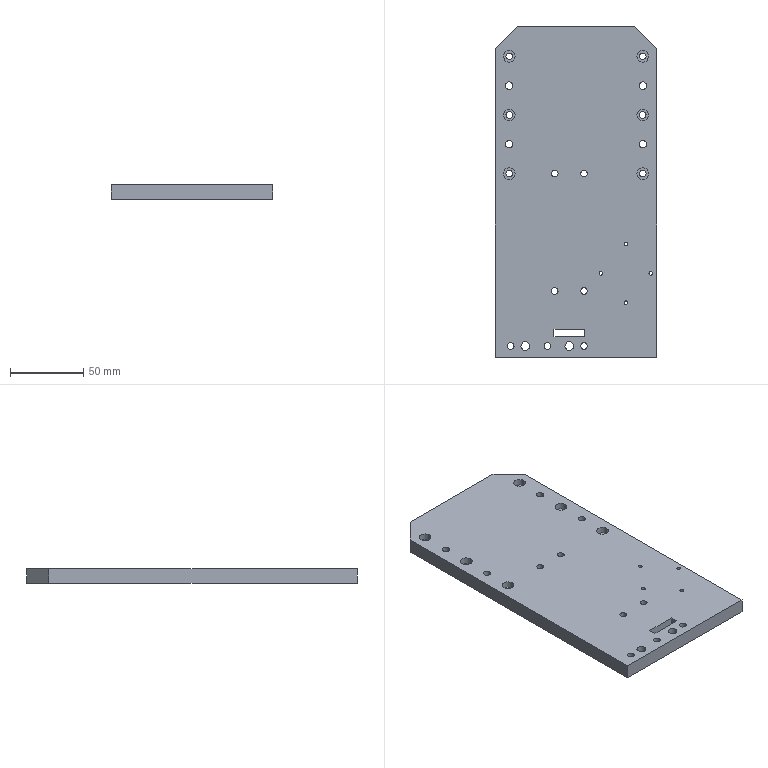Component | SolidWorks | GbgbYAxisConnectionPlate-1 | 1 solid | 97 faces | box 110 x 225 x 10 mm | volume 238530 mm3 | cylinder 72 | plane 25 | commonest cylinder face diameters 8 x26 4.5 x26 5 x8 2.5 x8 6 x4 | material AL6061
build123d program:
from build123d import *

# Parameters (mm, degrees)
SKETCH1_W                                            = 110
SKETCH1_H                                            = 220
BOSS_EXTRUDE1_DEPTH                                  = 5
M3_TAPPED_HOLE1_D                                    = 2.5
HOLE_SIZE_ACCORDING_TO_THE_TYPE_OF_HEX_S_D           = 4.5
HOLE_SIZE_ACCORDING_TO_THE_TYPE_OF_HEX_S_CBORE_D     = 8
HOLE_SIZE_ACCORDING_TO_THE_TYPE_OF_HEX_S_CBORE_DEPTH = 4.6
LPATTERN1_COUNT                                      = 3
LPATTERN1_PITCH                                      = 40
SKETCH13_W                                           = 21
SKETCH13_H                                           = 5
CUT_EXTRUDE2_DEPTH                                   = 10
MOVE_FACE1_BY                                        = 5
HOLE_SIZE_ACCORDING_TO_THE_TYPE_OF_H_2_D             = 4.5
HOLE_SIZE_ACCORDING_TO_THE_TYPE_OF_H_2_CBORE_D       = 8
HOLE_SIZE_ACCORDING_TO_THE_TYPE_OF_H_2_CBORE_DEPTH   = 4.6
HOLE_SIZE_ACCORDING_TO_THE_TYPE_OF_H_3_D             = 4.5
HOLE_SIZE_ACCORDING_TO_THE_TYPE_OF_H_3_CBORE_D       = 8
HOLE_SIZE_ACCORDING_TO_THE_TYPE_OF_H_3_CBORE_DEPTH   = 4.6
SKETCH20_R                                           = 3
CUT_EXTRUDE3_DEPTH                                   = 128.867
SKETCH21_R                                           = 2.5
CUT_EXTRUDE4_DEPTH                                   = 15
LPATTERN2_COUNT                                      = 2
LPATTERN2_PITCH                                      = 40
CHAMFER1_SIZE                                        = 15


with BuildPart() as part:
    # Sketch1 → Boss-Extrude1 (new, symmetric)
    with BuildSketch(Plane.XY):
        Rectangle(SKETCH1_W, SKETCH1_H)
    extrude(amount=BOSS_EXTRUDE1_DEPTH, both=True)

    # M3 Tapped Hole1 (through all)
    with Locations(Plane.XY.offset(5)):
        with Locations((34, -38), (17, -58), (51, -58), (34, -78)):
            Hole(M3_TAPPED_HOLE1_D / 2)

    # Hole Size according to the type of hex s (through all)
    with Locations(Plane.XY.offset(5)):
        with Locations((-45.5, 90), (45.5, 90)):
            hole_size_according_to_the_type_of_hex_s = CounterBoreHole(HOLE_SIZE_ACCORDING_TO_THE_TYPE_OF_HEX_S_D / 2, HOLE_SIZE_ACCORDING_TO_THE_TYPE_OF_HEX_S_CBORE_D / 2, HOLE_SIZE_ACCORDING_TO_THE_TYPE_OF_HEX_S_CBORE_DEPTH)

    # LPattern1: Hole Size according to the type of hex s ×3
    with Locations(*[(0, -i * LPATTERN1_PITCH, 0) for i in range(1, LPATTERN1_COUNT)]):
        add(hole_size_according_to_the_type_of_hex_s, mode=Mode.SUBTRACT)

    # Sketch13 → Cut-Extrude2 (cut)
    with BuildSketch(Plane(origin=(0, 0, -5), x_dir=(-1, 0, 0), z_dir=(0, 0, -1))):
        with Locations((4.5, -98.6)):
            Rectangle(SKETCH13_W, SKETCH13_H)
    extrude(amount=-CUT_EXTRUDE2_DEPTH, mode=Mode.SUBTRACT)

    # Move Face1: a face moved outward by 5.0
    extrude(part.faces().sort_by_distance((0, -110, 0))[0], amount=MOVE_FACE1_BY, dir=(0, -1, 0))

    # Hole Size according to the type of h 2 (through all)
    with Locations(Plane(origin=(0, 0, -5), x_dir=(-1, 0, 0), z_dir=(0, 0, -1))):
        with Locations((44.5, -107.5), (19.5, -107.5), (-5.5, -107.5)):
            CounterBoreHole(HOLE_SIZE_ACCORDING_TO_THE_TYPE_OF_H_2_D / 2, HOLE_SIZE_ACCORDING_TO_THE_TYPE_OF_H_2_CBORE_D / 2, HOLE_SIZE_ACCORDING_TO_THE_TYPE_OF_H_2_CBORE_DEPTH)

    # Hole Size according to the type of h 3 (through all)
    with Locations(Plane(origin=(0, 0, -5), x_dir=(-1, 0, 0), z_dir=(0, 0, -1))):
        with Locations((-5.5, -70), (14.5, -70), (-5.5, 10), (14.5, 10)):
            CounterBoreHole(HOLE_SIZE_ACCORDING_TO_THE_TYPE_OF_H_3_D / 2, HOLE_SIZE_ACCORDING_TO_THE_TYPE_OF_H_3_CBORE_D / 2, HOLE_SIZE_ACCORDING_TO_THE_TYPE_OF_H_3_CBORE_DEPTH)

    # Sketch20 → Cut-Extrude3 (cut, through all)
    with BuildSketch(Plane(origin=(0, 0, -5), x_dir=(-1, 0, 0), z_dir=(0, 0, -1))):
        with Locations((4.5, -107.5)):
            Circle(SKETCH20_R)
        with Locations((34.5, -107.5)):
            Circle(SKETCH20_R)
    extrude(amount=-CUT_EXTRUDE3_DEPTH, mode=Mode.SUBTRACT)

    # Sketch21 → Cut-Extrude4 (cut)
    with BuildSketch(Plane.XY.offset(5)):
        with Locations((-45.5, 70)):
            Circle(SKETCH21_R)
        with Locations((45.5, 70)):
            Circle(SKETCH21_R)
    cut_extrude4 = extrude(amount=-CUT_EXTRUDE4_DEPTH, mode=Mode.SUBTRACT)

    # LPattern2: Cut-Extrude4 ×2
    with Locations(*[(0, -i * LPATTERN2_PITCH, 0) for i in range(1, LPATTERN2_COUNT)]):
        add(cut_extrude4, mode=Mode.SUBTRACT)

    # Chamfer1
    chamfer1_edges = [part.edges().sort_by_distance(p)[0] for p in [
        (-55, 110, 0),
        (55, 110, 0),
    ]]
    chamfer(chamfer1_edges, length=CHAMFER1_SIZE)


solid = part.part

# Placed as in the assembly
solid = solid.moved(Location((84.946, 484.94, 385.232), (0, 0, 0)))